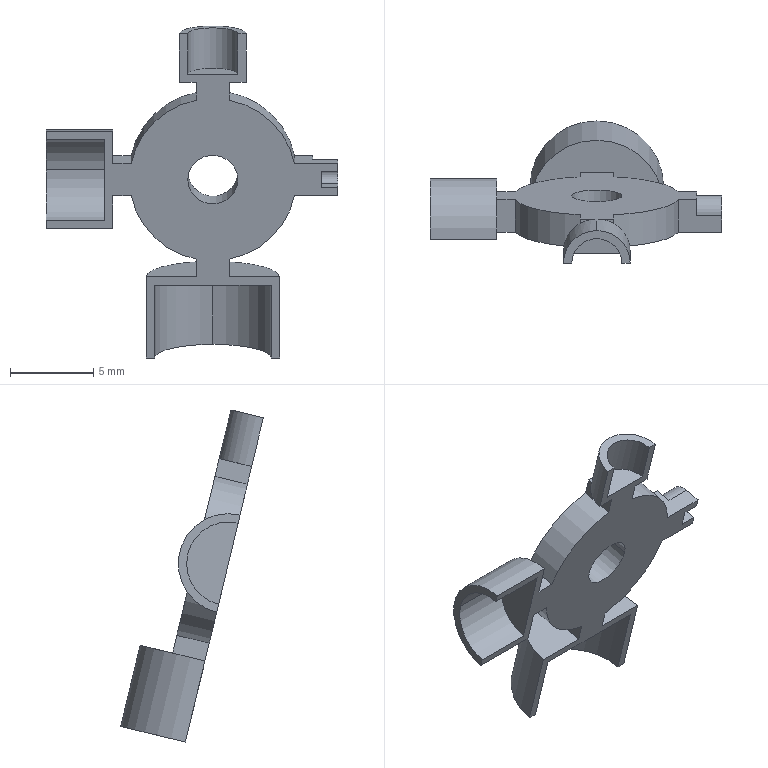Component | SolidWorks | SeedingAssemblyA-1_SeedSpoonPlate-1 | 1 solid | 46 faces | box 17.5 x 8.56 x 19.91 mm | volume 235 mm3 | plane 28 | cylinder 18 | commonest cylinder face diameters 10 x4 3 x3 2 x2 4 x2 5 x2 7 x2 8 x1 6 x1
build123d program:
from build123d import *

# Parameters (mm, degrees)
BOSS_EXTRUDE1_DEPTH = 2
SKETCH2_R           = 1.5
CUT_EXTRUDE1_DEPTH  = 2
BOSS_EXTRUDE2_DEPTH = 5
SKETCH4_R           = 3.5
CUT_EXTRUDE2_DEPTH  = 4.5
BOSS_EXTRUDE3_DEPTH = 4
CUT_EXTRUDE3_DEPTH  = 3.5
BOSS_EXTRUDE4_DEPTH = 3
CUT_EXTRUDE4_DEPTH  = 2.5
BOSS_EXTRUDE5_DEPTH = 1.5
CUT_EXTRUDE5_DEPTH  = 1


with BuildPart() as part:
    # Sketch1 → Boss-Extrude1 (new body)
    with BuildSketch(Plane.XY):
        with BuildLine():
            Line((6, -1), (6, 1))
            Line((6, 1), (4.899, 1))
            ThreePointArc((4.899, 1), (3.536, 3.536), (1, 4.899))
            Line((1, 4.899), (1, 6))
            Line((1, 6), (-1, 6))
            Line((-1, 6), (-1, 4.899))
            ThreePointArc((-1, 4.899), (-3.536, 3.536), (-4.899, 1))
            Line((-4.899, 1), (-6, 1))
            Line((-6, 1), (-6, -1))
            Line((-6, -1), (-4.899, -1))
            ThreePointArc((-4.899, -1), (-3.536, -3.536), (-1, -4.899))
            Line((-1, -4.899), (-1, -6))
            Line((-1, -6), (1, -6))
            Line((1, -6), (1, -4.899))
            ThreePointArc((1, -4.899), (3.536, -3.536), (4.899, -1))
            Line((4.899, -1), (6, -1))
        make_face()
    extrude(amount=BOSS_EXTRUDE1_DEPTH)

    # Sketch2 → Cut-Extrude1 (cut)
    with BuildSketch(Plane(origin=(0, 0, 0), x_dir=(-1, 0, 0), z_dir=(0, 0, -1))):
        Circle(SKETCH2_R)
    extrude(amount=-CUT_EXTRUDE1_DEPTH, mode=Mode.SUBTRACT)

    # Sketch3 → Boss-Extrude2 (add)
    with BuildSketch(Plane(origin=(0, 6, 0), x_dir=(1, 0, 0), z_dir=(0, 1, 0))):
        with BuildLine():
            Line((-4, 0), (4, 0))
            ThreePointArc((4, 0), (0, -4), (-4, 0))
        make_face()
    extrude(amount=BOSS_EXTRUDE2_DEPTH)

    # Sketch4 → Cut-Extrude2 (cut)
    with BuildSketch(Plane(origin=(0, 11, 0), x_dir=(1, 0, 0), z_dir=(0, 1, 0))):
        Circle(SKETCH4_R)
    extrude(amount=-CUT_EXTRUDE2_DEPTH, mode=Mode.SUBTRACT)

    # Sketch6 → Boss-Extrude3 (add)
    with BuildSketch(Plane.ZY.offset(6)):
        with BuildLine():
            Line((0, 3), (0, -3))
            ThreePointArc((0, -3), (3, 0), (0, 3))
        make_face()
    extrude(amount=BOSS_EXTRUDE3_DEPTH)

    # Sketch7 → Cut-Extrude3 (cut)
    with BuildSketch(Plane.ZY.offset(10)):
        with BuildLine():
            Line((0, 2.5), (0, -2.5))
            ThreePointArc((0, -2.5), (2.5, 0), (0, 2.5))
        make_face()
    extrude(amount=-CUT_EXTRUDE3_DEPTH, mode=Mode.SUBTRACT)

    # Sketch8 → Boss-Extrude4 (add)
    with BuildSketch(Plane.XZ.offset(6)):
        with BuildLine():
            Line((-2, 0), (2, 0))
            ThreePointArc((2, 0), (0, 2), (-2, 0))
        make_face()
    extrude(amount=BOSS_EXTRUDE4_DEPTH)

    # Sketch9 → Cut-Extrude4 (cut)
    with BuildSketch(Plane(origin=(0, -9, 0), x_dir=(-1, 0, 0), z_dir=(0, -1, 0))):
        with BuildLine():
            Line((-1.5, 0), (1.5, 0))
            ThreePointArc((1.5, 0), (0, -1.5), (-1.5, 0))
        make_face()
    extrude(amount=-CUT_EXTRUDE4_DEPTH, mode=Mode.SUBTRACT)

    # Sketch10 → Boss-Extrude5 (add)
    with BuildSketch(Plane(origin=(6, 0, 0), x_dir=(0, 0, -1), z_dir=(1, 0, 0))):
        with BuildLine():
            Line((-1, 1), (0, 1))
            Line((0, 1), (0, -1))
            Line((0, -1), (-1, -1))
            ThreePointArc((-1, -1), (-2, 0), (-1, 1))
        make_face()
    extrude(amount=BOSS_EXTRUDE5_DEPTH)

    # Sketch11 → Cut-Extrude5 (cut)
    with BuildSketch(Plane(origin=(7.5, 0, 0), x_dir=(0, 0, -1), z_dir=(1, 0, 0))):
        with BuildLine():
            Line((-0.5, 0.5), (0, 0.5))
            Line((0, 0.5), (0, -0.5))
            Line((0, -0.5), (-0.5, -0.5))
            Line((-0.5, -0.5), (-1, -0.5))
            ThreePointArc((-1, -0.5), (-1.5, 0), (-1, 0.5))
            Line((-1, 0.5), (-0.5, 0.5))
        make_face()
    extrude(amount=-CUT_EXTRUDE5_DEPTH, mode=Mode.SUBTRACT)


solid = part.part

# Placed as in the assembly
solid = solid.moved(Location((90.731, -277.11, -267.803), (-76.497, 0, 0)))